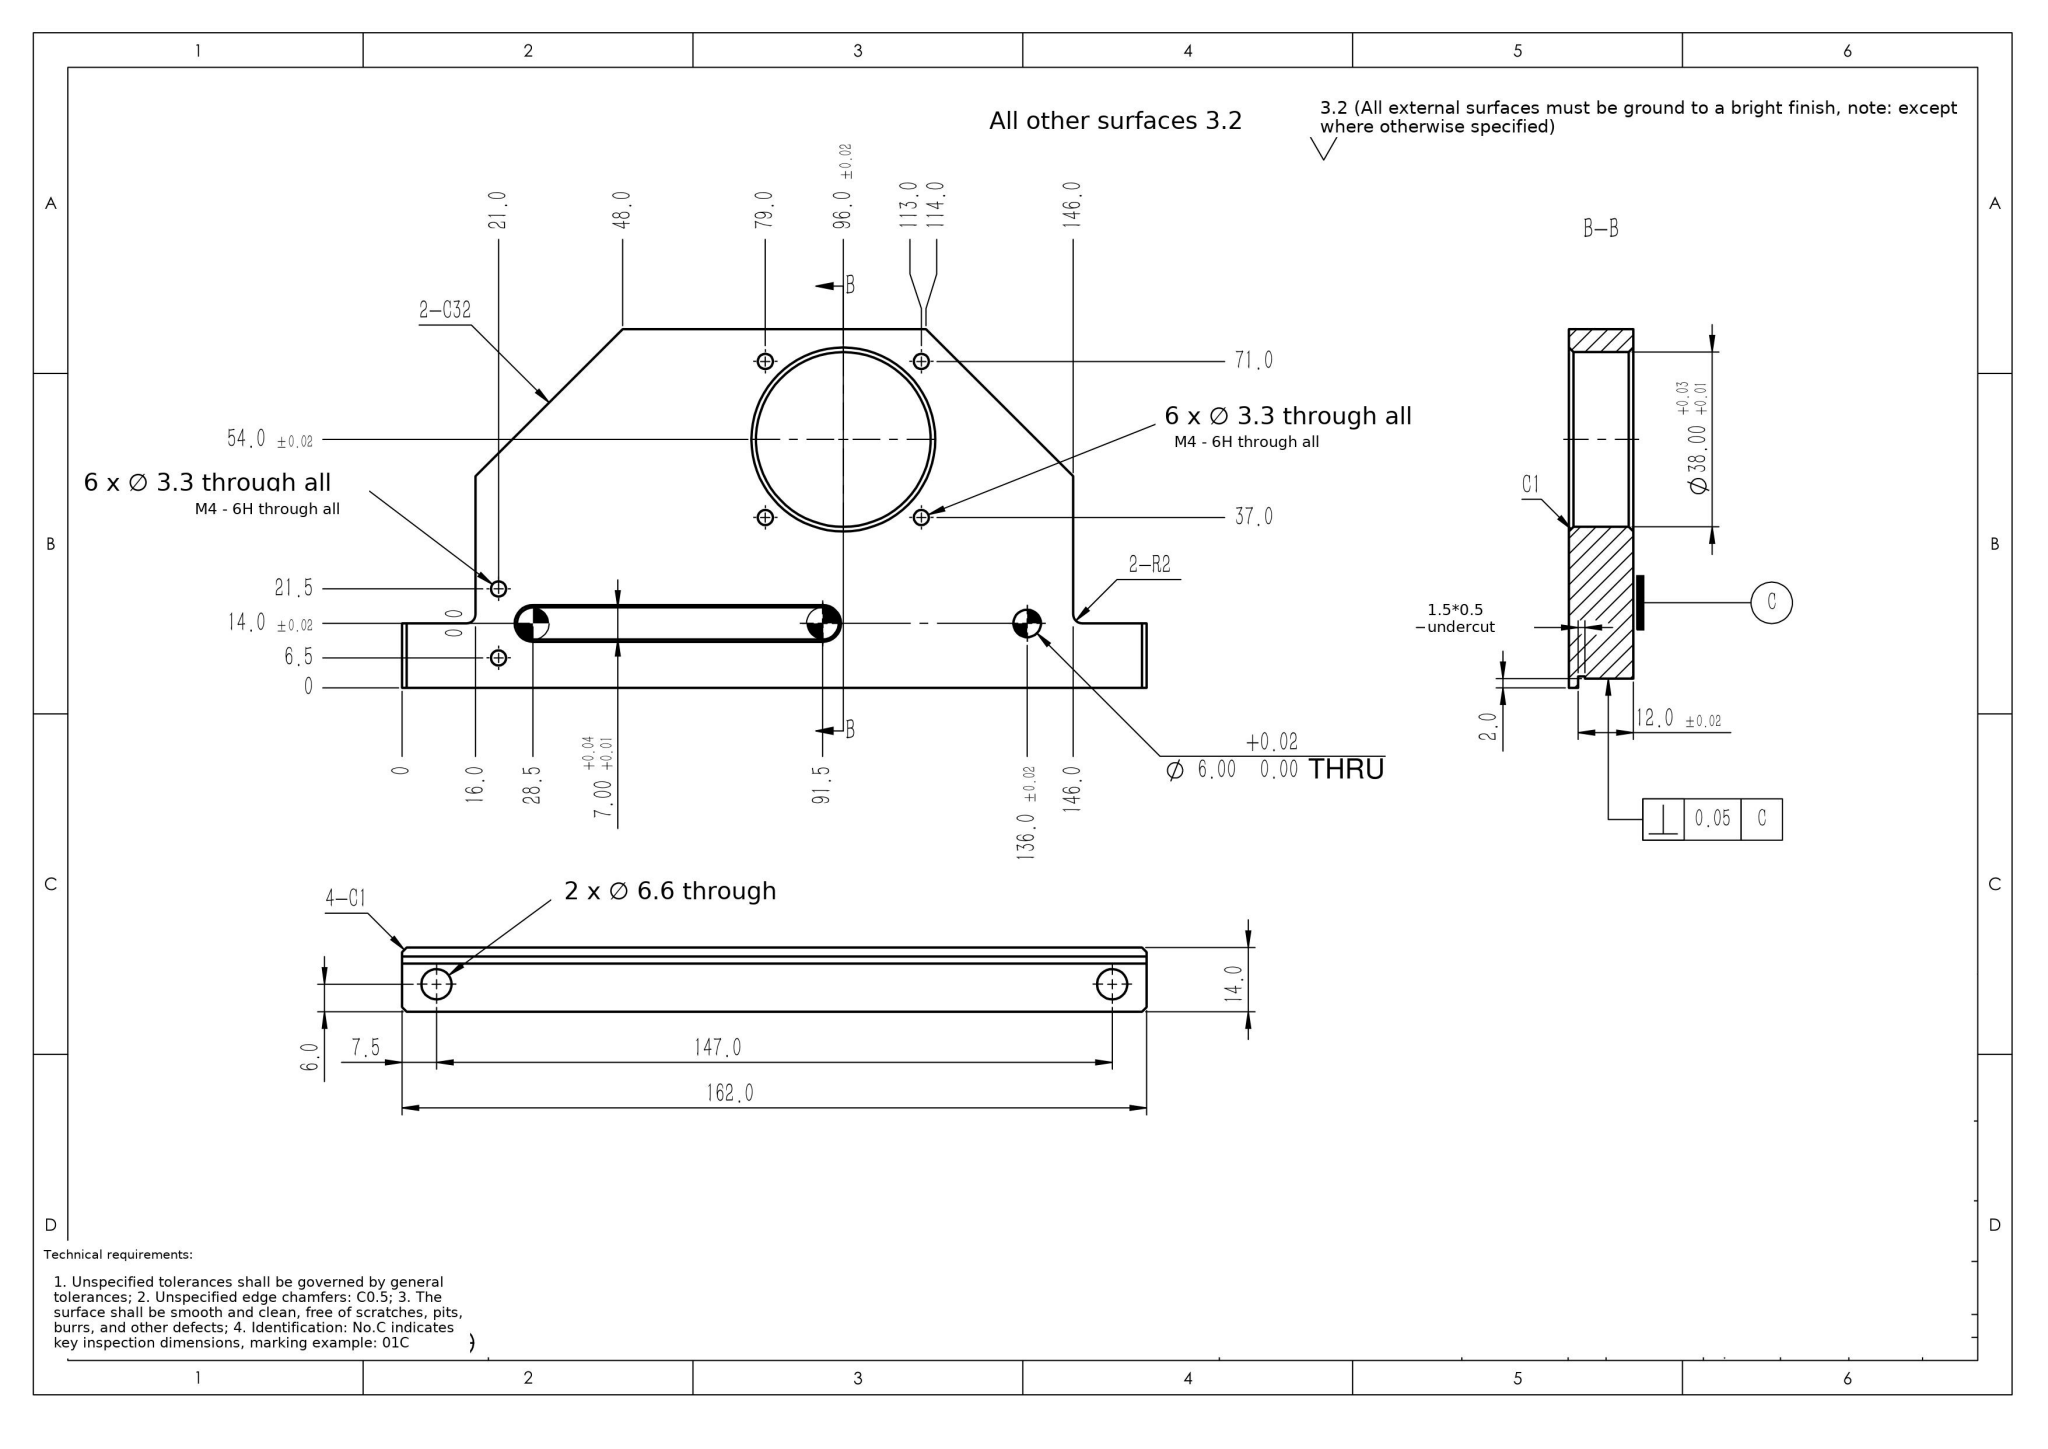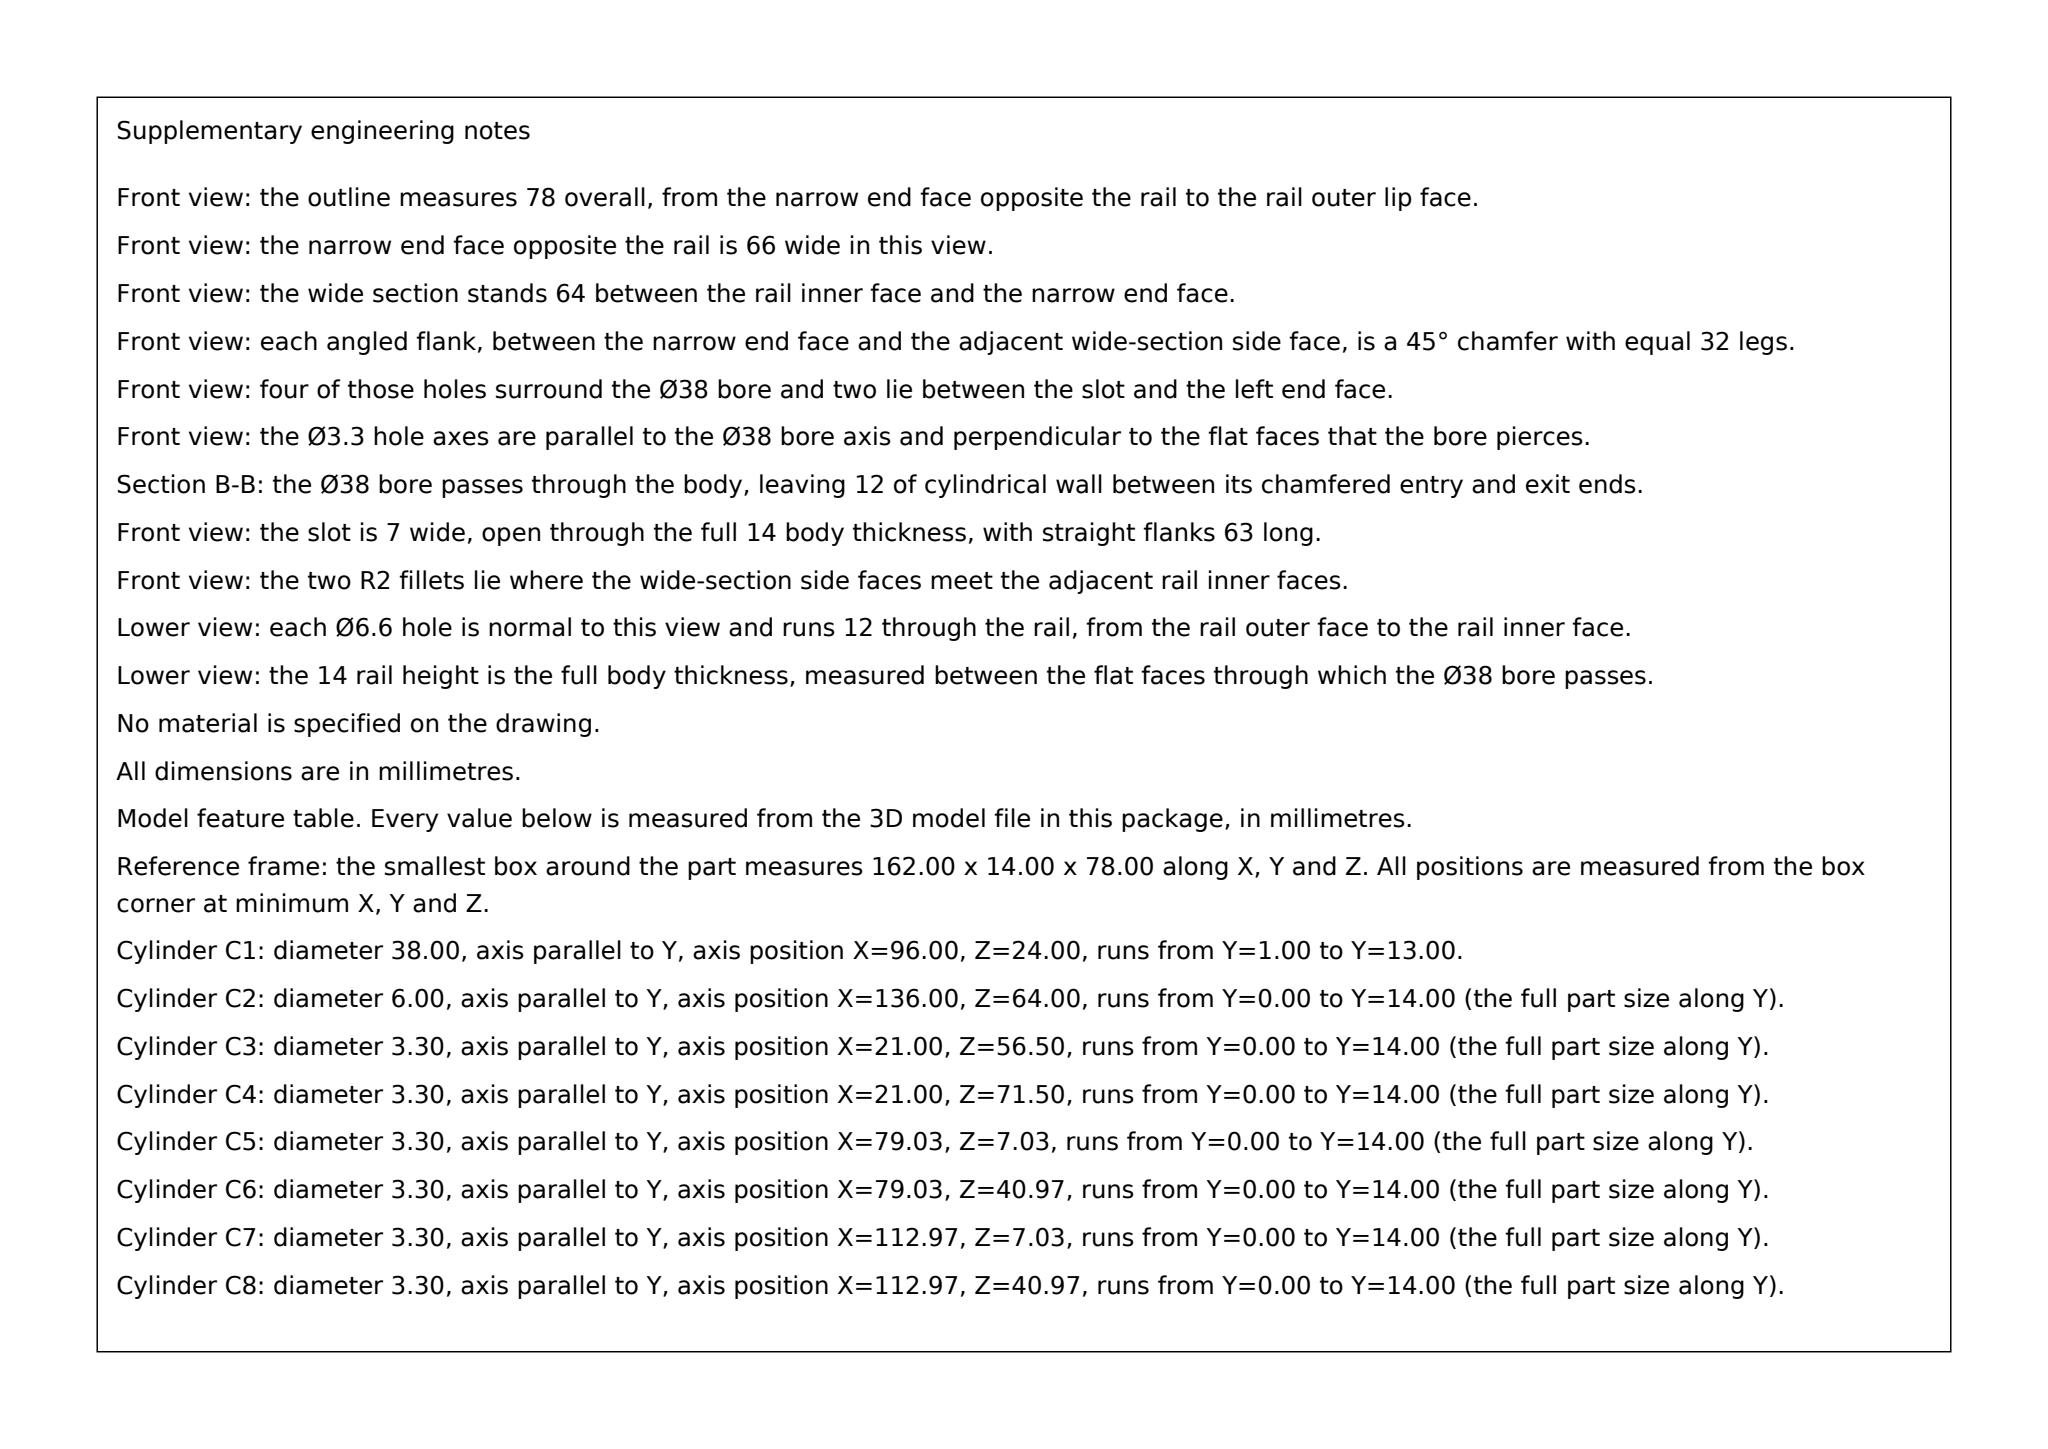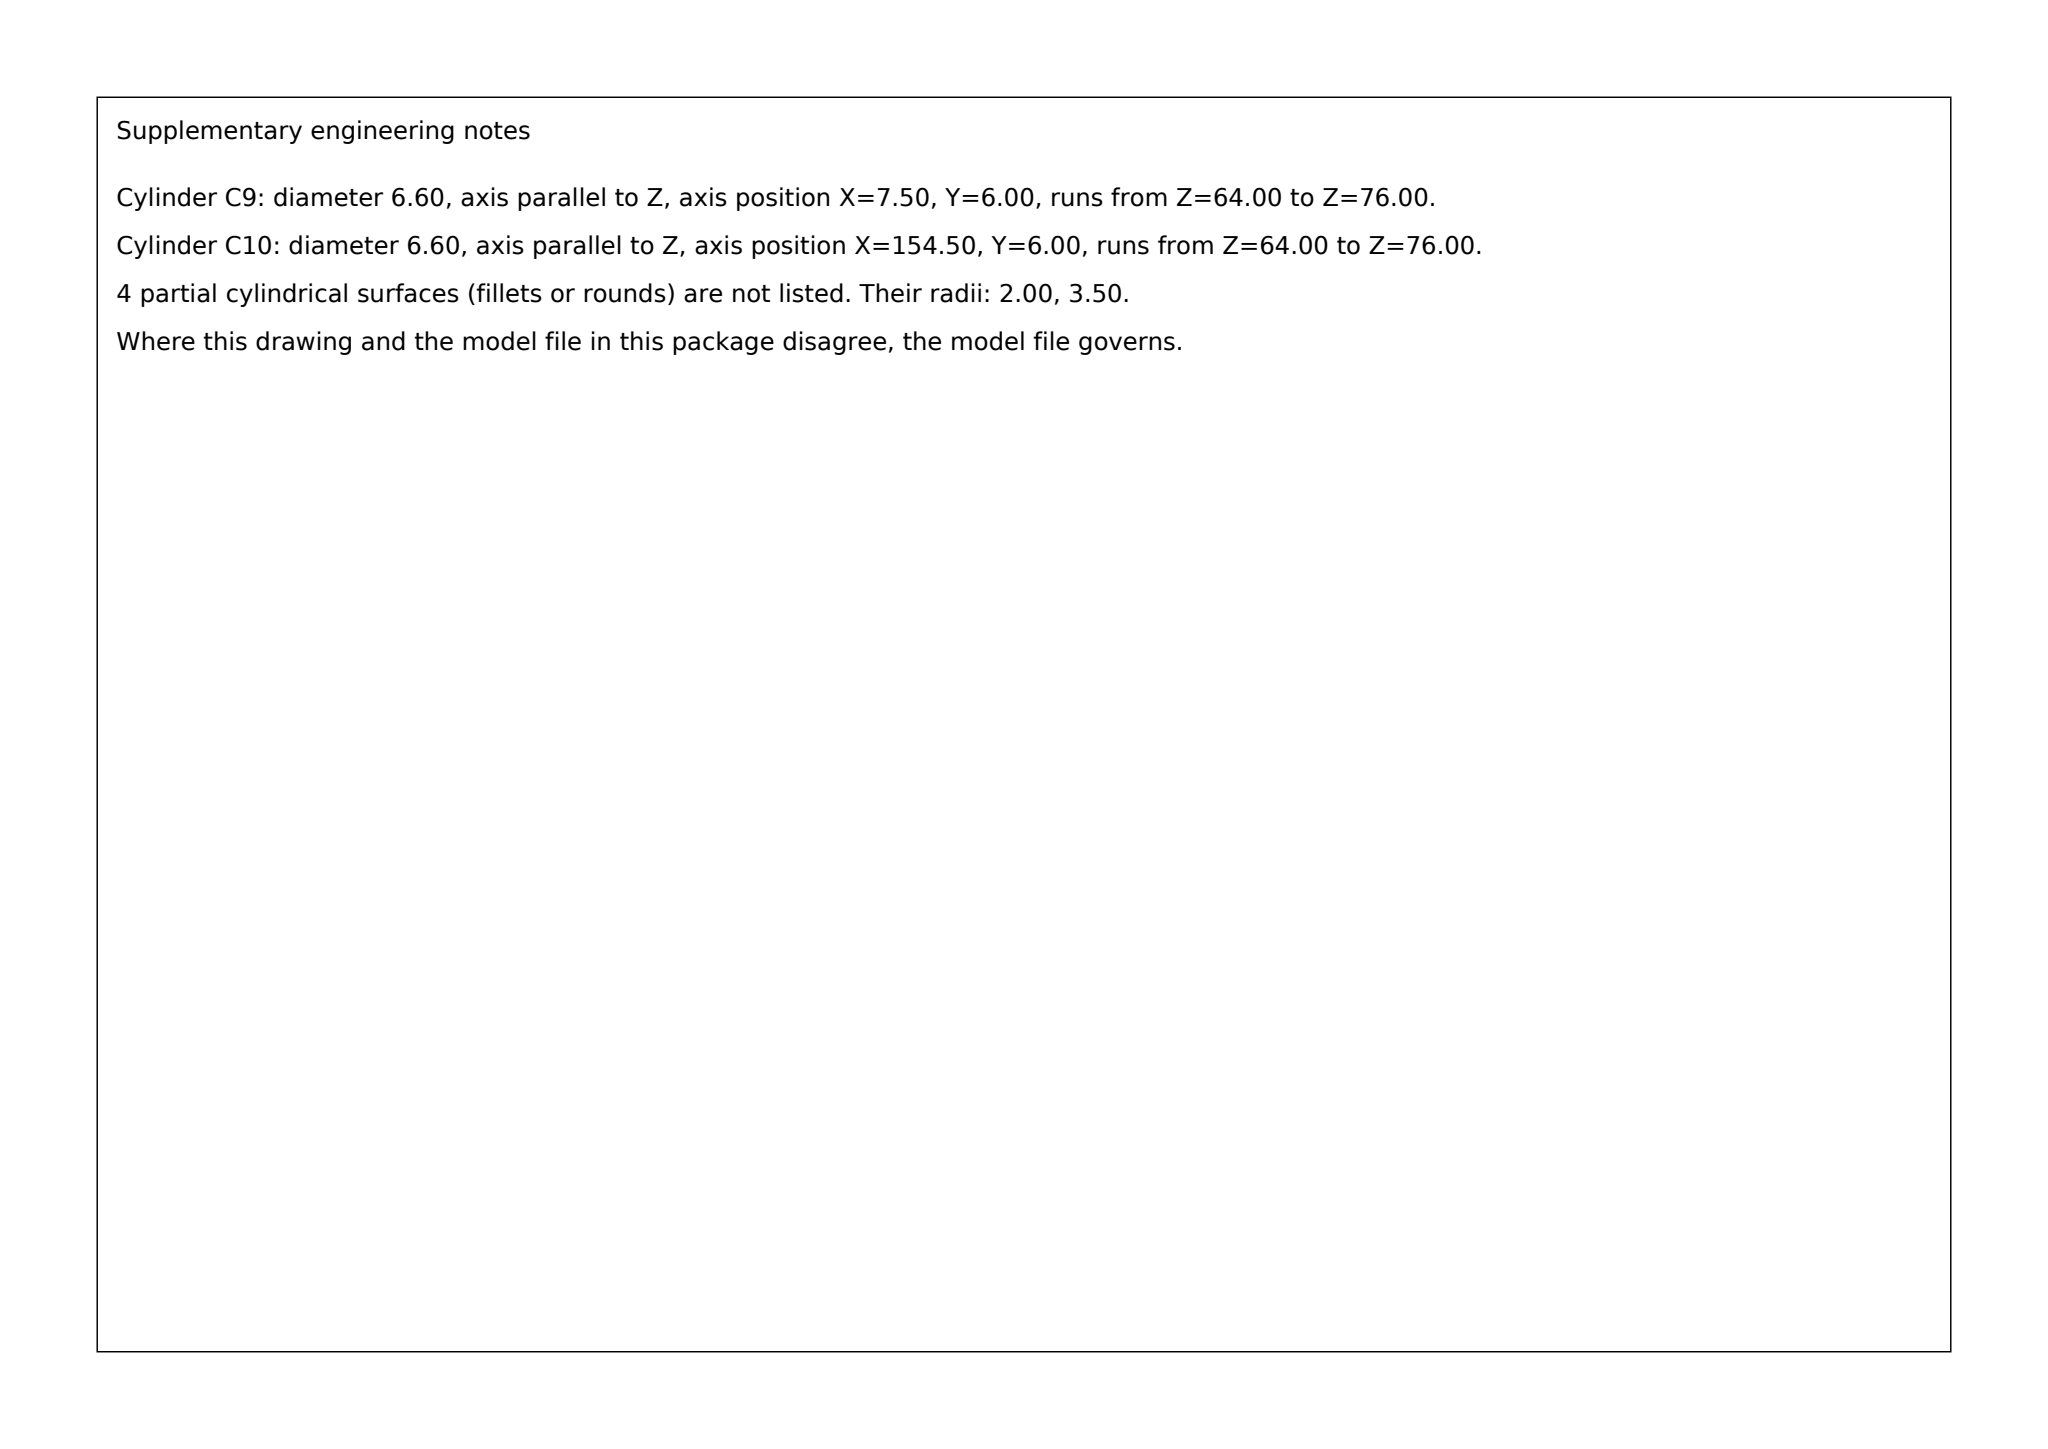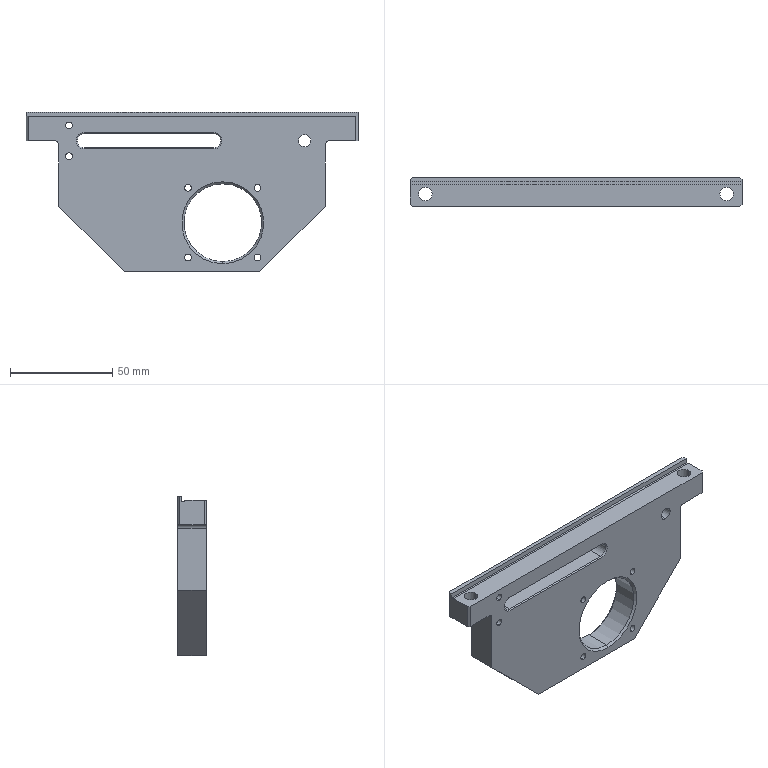Part | SolidWorks | mm | 1 solid | 58 faces | box 162 x 14 x 78 mm | volume 105200 mm3 | plane 26 | cylinder 24 | cone 8 | commonest cylinder face diameters 3.3 x12 6.6 x4 6 x2 38 x2 7 x2 4 x2
Drawing notes:
FRONT VIEW: OVERALL HT 78.0; 2-C32 BEGINS 46.0 ABOVE BOTTOM | from the solid: bbox_xyz Z=78.0; top face plane z=78 with vertical planes x=16.0 & x=146.0; 32x32 chamfer => 78-32=46.0 above bottom
SLOT Ø7.00 (+0.04/+0.01) WIDE, END CENTERS X=28.5 & X=91.5, Z=64.0 FROM BOTTOM: THRU 14.0 THK PLATE (Y=0 TO Y=14.0) | from the solid: Ø7.0 slot-end arcs (y axis) at X=28.5 and X=91.5, Z=64.0 run y=0.5 to 13.5; slot walls z=60.5 and z=67.5 extend y=0.5-13.5; 0.5 chamfer faces/cones exist at BOTH y=0-0.5 and y=13.5-14.0, so the slot opens on both faces of the 14.0 thk plate (no blind bottom face).
BOTH SLOT ENDS: CHAMFER 0.5 X 45° AT MOUTH (Ø7.0 TO Ø8.0, 90° INCL) ON BOTH FACES Y=0 AND Y=14.0 | from the solid: Cones 90° incl at slot ends appear at y=13.5-14.0 (ref Ø7.0) and y=0.0-0.5 (ref Ø8.0), X=24.5/91.5, Z=60-68; matching 45° inclined planes at y=0-0.5 and y=13.5-14.0 along x=28.5-91.5.
END STEP FACES (X=0-14.0 & X=148.0-162.0) AT Z=64.0 FROM BOTTOM FACE Z=0, i.e. 14.0 BELOW TOP FACE Z=78.0; END FACES X=0 & X=162.0 RUN Z=64.0 TO 78.0 | from the solid: axis_planes z offset 64.0 extents x[0,14] and x[148,162] y[0,14]; planes x=0.0 and x=162.0 extent z[64,78]
2X Ø6.6 DP 12.0 INTO END STEP FACES (Z=64.0 TO Z=76.0), AT X=7.5 & X=154.5, Y=6.0 | from the solid: cylinders hole/bore dia 6.6 axis z at (7.5,6.0) and (154.5,6.0), from 64.0 to 76.0
2X R2.0 FILLET, FULL 14.0 THK (Y=0 TO 14.0), CENTERS X=14.0 & X=148.0, Z=62.0, BLENDING STEP FACE Z=64.0 TO WALLS X=16.0 & X=146.0 | from the solid: concave arc dia 4.0 axis y at (14.0,-,62.0) and (148.0,-,62.0), from y=0.0 to 14.0, arc 90°